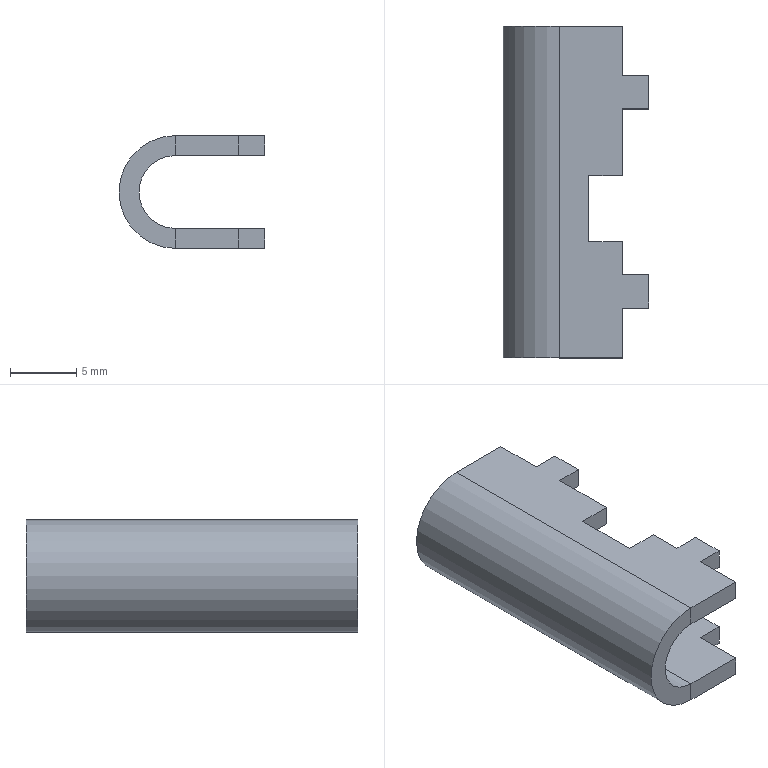Component | SolidWorks | AEBox-DoorHinge-2 | 1 solid | 39 faces | volume 760 mm3 | plane 36 | cylinder 3 | commonest cylinder face diameters 5.5 x1 8.5 x1 2.4 x1